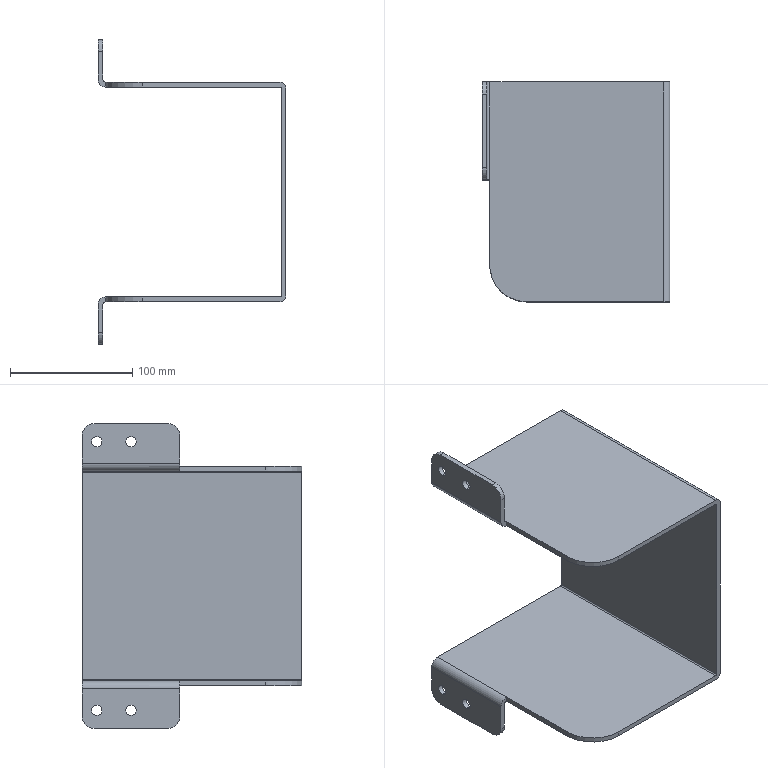Component | SolidWorks | 000-08-1 | 1 solid | 40 faces | box 154 x 180 x 250 mm | volume 357001 mm3 | cylinder 22 | plane 18 | commonest cylinder face diameters 8.5 x8 20 x4 13 x2 2 x2 5 x2 10 x2 60 x2 | material Transparent Acrylic
build123d program:
from build123d import *

# Parameters (mm, degrees)
EXTRUDE_THIN1_DEPTH = 90
SKETCH2_W           = 6.39
SKETCH2_H           = 100
CUT_EXTRUDE1_DEPTH  = 308.109
FILLET1_R           = 30
SKETCH3_R           = 4.25
CUT_EXTRUDE2_DEPTH  = 216
FILLET2_R           = 10


with BuildPart() as part:
    # Sketch1 → Extrude-Thin1 (new, symmetric)
    with BuildSketch(Plane(origin=(0, 0, 0), x_dir=(1, 0, 0), z_dir=(0, 1, 0))):
        with BuildLine():
            Line((-125, 150), (-92.5, 150))
            ThreePointArc((-92.5, 150), (-90.732, 149.268), (-90, 147.5))
            Line((-90, 147.5), (-90, 5))
            ThreePointArc((-90, 5), (-88.536, 1.464), (-85, 0))
            Line((-85, 0), (85, 0))
            ThreePointArc((85, 0), (88.536, 1.464), (90, 5))
            Line((90, 5), (90, 147.5))
            ThreePointArc((90, 147.5), (90.732, 149.268), (92.5, 150))
            Line((92.5, 150), (125, 150))
            Line((125, 150), (125, 154))
            Line((125, 154), (92.5, 154))
            ThreePointArc((92.5, 154), (87.904, 152.096), (86, 147.5))
            Line((86, 147.5), (86, 5))
            ThreePointArc((86, 5), (85.707, 4.293), (85, 4))
            Line((85, 4), (-85, 4))
            ThreePointArc((-85, 4), (-85.707, 4.293), (-86, 5))
            Line((-86, 5), (-86, 147.5))
            ThreePointArc((-86, 147.5), (-87.904, 152.096), (-92.5, 154))
            Line((-92.5, 154), (-125, 154))
            Line((-125, 154), (-125, 150))
        make_face()
    extrude(amount=EXTRUDE_THIN1_DEPTH, both=True)

    # Sketch2 → Cut-Extrude1 (cut, through all)
    with BuildSketch(Plane(origin=(125, 0, 0), x_dir=(0, 0, -1), z_dir=(1, 0, 0))):
        with Locations((150.805, -40)):
            Rectangle(SKETCH2_W, SKETCH2_H)
    extrude(amount=-CUT_EXTRUDE1_DEPTH, mode=Mode.SUBTRACT)

    # Fillet1
    fillet1_edges = [part.edges().sort_by_distance(p)[0] for p in [
        (-88.002, -90, -147.61),
        (88.002, -90, -147.61),
    ]]
    fillet(fillet1_edges, radius=FILLET1_R)

    # Sketch3 → Cut-Extrude2 (cut, through all)
    with BuildSketch(Plane.XY.offset(-150)):
        with Locations((-110, 78)):
            Circle(SKETCH3_R)
        with Locations((-110, 50)):
            Circle(SKETCH3_R)
        with Locations((110, 78)):
            Circle(SKETCH3_R)
        with Locations((110, 50)):
            Circle(SKETCH3_R)
    extrude(amount=-CUT_EXTRUDE2_DEPTH, mode=Mode.SUBTRACT)

    # Fillet2
    fillet2_edges = [part.edges().sort_by_distance(p)[0] for p in [
        (-125, 90, -152),
        (-125, 10, -152),
        (125, 10, -152),
        (125, 90, -152),
    ]]
    fillet(fillet2_edges, radius=FILLET2_R)


solid = part.part

# Placed as in the assembly
solid = solid.moved(Location((333, 721, 0), (0, 90, 0)))